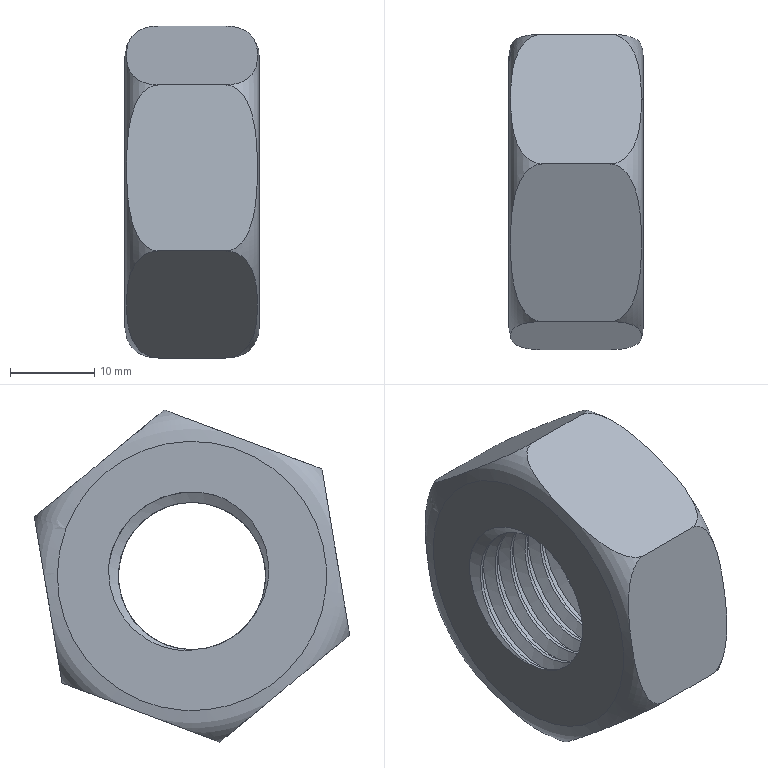Component | NX | CCJ-016_2 | 1 solid | 15 faces | volume 11973 mm3 | plane 9 | cylinder 2 | torus 2 | spline 2 | commonest cylinder face diameters 17.5 x1 20 x1